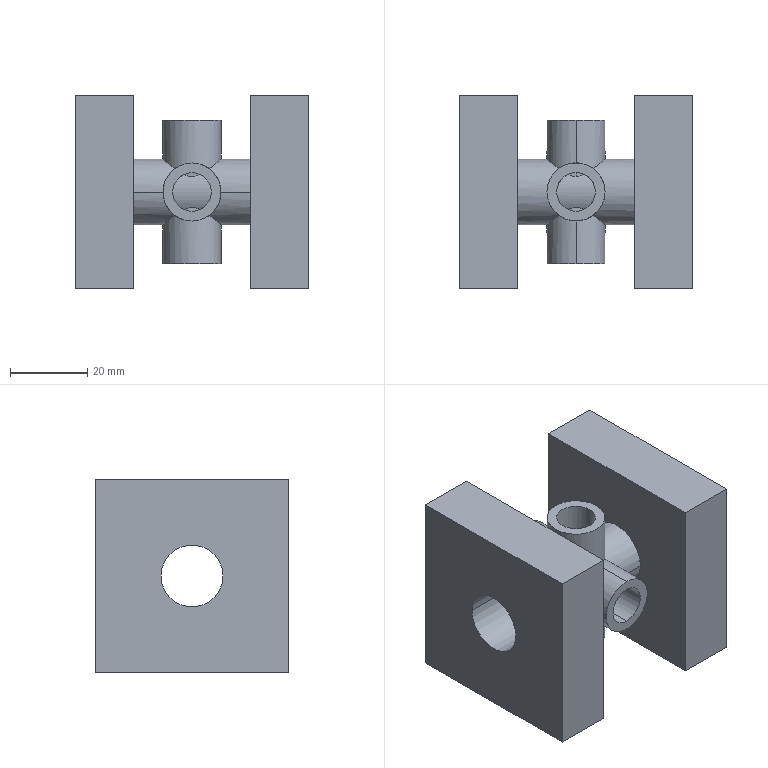Component | SolidWorks | OuterFlipShell-1 | 1 solid | 53 faces | volume 74126 mm3 | cylinder 37 | plane 16 | commonest cylinder face diameters 15 x18 17 x9 10 x8 16 x2